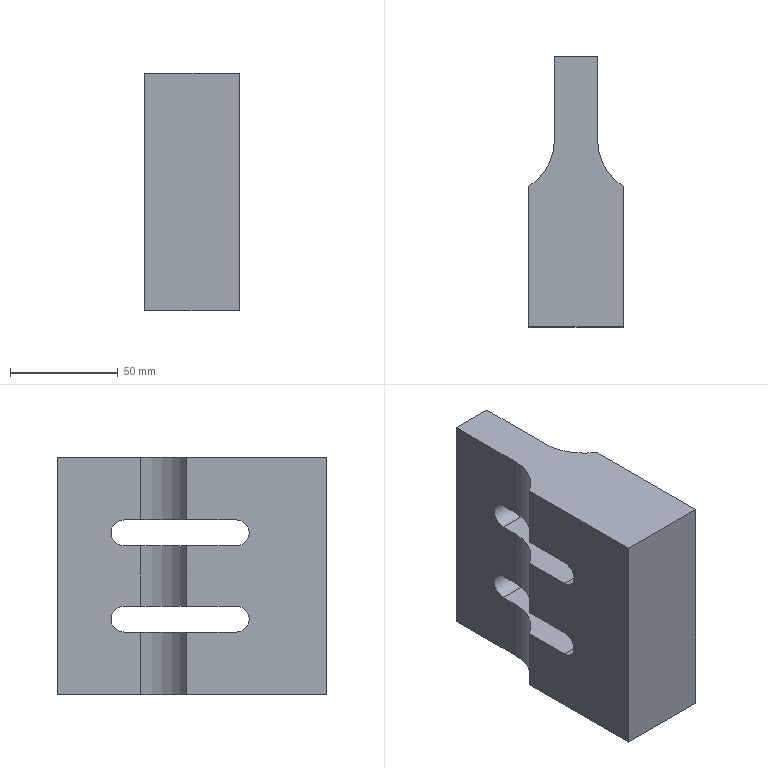Component | SolidWorks | Assembly4.1-1_113.1-1 | 1 solid | 22 faces | box 44 x 125 x 110 mm | volume 414066 mm3 | plane 12 | cylinder 10 | commonest cylinder face diameters 50 x6 12 x4
build123d program:
from build123d import *

# Parameters (mm, degrees)
SKETCH1_W           = 110
SKETCH1_H           = 125
BOSS_EXTRUDE1_DEPTH = 22
CUT_EXTRUDE1_DEPTH  = 124
CUT_EXTRUDE2_DEPTH  = 62


with BuildPart() as part:
    # Sketch1 → Boss-Extrude1 (new, symmetric)
    with BuildSketch(Plane.XY):
        Rectangle(SKETCH1_W, SKETCH1_H)
    extrude(amount=BOSS_EXTRUDE1_DEPTH, both=True)

    # Sketch2 → Cut-Extrude1 (cut)
    with BuildSketch(Plane(origin=(55, 0, 0), x_dir=(0, 0, -1), z_dir=(1, 0, 0))):
        with BuildLine():
            Line((-22, 2.5), (-46.846, 2.5))
            Line((-46.846, 2.5), (-46.846, 62.5))
            Line((-46.846, 62.5), (-10, 62.5))
            Line((-10, 62.5), (-10, 23.854))
            ThreePointArc((-10, 23.854), (-13.206, 11.607), (-22, 2.5))
        make_face()
        with BuildLine():
            Line((46.846, 62.5), (10, 62.5))
            Line((10, 62.5), (10, 23.854))
            ThreePointArc((10, 23.854), (13.206, 11.607), (22, 2.5))
            Line((22, 2.5), (46.846, 2.5))
            Line((46.846, 2.5), (46.846, 62.5))
        make_face()
    extrude(amount=-CUT_EXTRUDE1_DEPTH, mode=Mode.SUBTRACT)

    # Sketch3 → Cut-Extrude2 (cut, symmetric)
    with BuildSketch(Plane.XY):
        with BuildLine():
            Line((-14, 31.5), (-14, -20.5))
            ThreePointArc((-14, -20.5), (-20, -26.5), (-26, -20.5))
            Line((-26, -20.5), (-26, 31.5))
            ThreePointArc((-26, 31.5), (-20, 37.5), (-14, 31.5))
        make_face()
        with BuildLine():
            Line((26, 31.5), (26, -20.5))
            ThreePointArc((26, -20.5), (20, -26.5), (14, -20.5))
            Line((14, -20.5), (14, 31.5))
            ThreePointArc((14, 31.5), (20, 37.5), (26, 31.5))
        make_face()
    extrude(amount=CUT_EXTRUDE2_DEPTH, both=True, mode=Mode.SUBTRACT)


solid = part.part

# Placed as in the assembly
solid = solid.moved(Location((0, 88, -0.4), (0, 90, 0)))
STEP:
#1=COLOUR_RGB('',0.7922,0.8196,0.9333);
#2=FILL_AREA_STYLE_COLOUR('',#1);
#3=FILL_AREA_STYLE('',(#2));
#4=SURFACE_STYLE_FILL_AREA(#3);
#5=SURFACE_SIDE_STYLE('',(#4));
#6=SURFACE_STYLE_USAGE(.BOTH.,#5);
#7=PRESENTATION_STYLE_ASSIGNMENT((#6));
#8=CARTESIAN_POINT('',(-0.3937,4.404,1.008));
#9=VERTEX_POINT('',#8);
#10=CARTESIAN_POINT('',(-0.3937,4.404,2.15));
#11=VERTEX_POINT('',#10);
#12=CARTESIAN_POINT('',(-0.3937,4.404,-2.732));
#13=DIRECTION('',(-0.,0.,1.));
#14=VECTOR('',#13,39.37);
#15=LINE('',#12,#14);
#16=EDGE_CURVE('',#9,#11,#15,.T.);
#17=ORIENTED_EDGE('',*,*,#16,.F.);
#18=CARTESIAN_POINT('',(-0.8661,3.563,1.008));
#19=VERTEX_POINT('',#18);
#20=CARTESIAN_POINT('',(-1.378,4.404,1.008));
#21=DIRECTION('',(0.,-0.,-1.));
#22=DIRECTION('',(0.,1.,-0.));
#23=AXIS2_PLACEMENT_3D('',#20,#21,#22);
#24=CIRCLE('',#23,0.9843);
#25=EDGE_CURVE('',#9,#19,#24,.T.);
#26=ORIENTED_EDGE('',*,*,#25,.T.);
#27=CARTESIAN_POINT('',(-0.8661,3.563,2.15));
#28=VERTEX_POINT('',#27);
#29=CARTESIAN_POINT('',(-0.8661,3.563,2.15));
#30=DIRECTION('',(-0.,0.,1.));
#31=VECTOR('',#30,39.37);
#32=LINE('',#29,#31);
#33=EDGE_CURVE('',#19,#28,#32,.T.);
#34=ORIENTED_EDGE('',*,*,#33,.T.);
#35=CARTESIAN_POINT('',(-1.378,4.404,2.15));
#36=DIRECTION('',(-0.,0.,1.));
#37=DIRECTION('',(0.,-1.,0.));
#38=AXIS2_PLACEMENT_3D('',#35,#36,#37);
#39=CIRCLE('',#38,0.9843);
#40=EDGE_CURVE('',#28,#11,#39,.T.);
#41=ORIENTED_EDGE('',*,*,#40,.T.);
#42=EDGE_LOOP('',(#17,#26,#34,#41));
#43=FACE_OUTER_BOUND('',#42,.T.);
#44=CARTESIAN_POINT('',(-1.378,4.404,-2.732));
#45=DIRECTION('',(-0.,0.,1.));
#46=DIRECTION('',(0.,1.,0.));
#47=AXIS2_PLACEMENT_3D('',#44,#45,#46);
#48=CYLINDRICAL_SURFACE('',#47,0.9843);
#49=ADVANCED_FACE('',(#43),#48,.F.);
#50=CARTESIAN_POINT('',(0.8661,3.563,1.008));
#51=VERTEX_POINT('',#50);
#52=CARTESIAN_POINT('',(0.8661,3.563,2.15));
#53=VERTEX_POINT('',#52);
#54=CARTESIAN_POINT('',(0.8661,3.563,-2.732));
#55=DIRECTION('',(-0.,0.,1.));
#56=VECTOR('',#55,39.37);
#57=LINE('',#54,#56);
#58=EDGE_CURVE('',#51,#53,#57,.T.);
#59=ORIENTED_EDGE('',*,*,#58,.F.);
#60=CARTESIAN_POINT('',(0.3937,4.404,1.008));
#61=VERTEX_POINT('',#60);
#62=CARTESIAN_POINT('',(1.378,4.404,1.008));
#63=DIRECTION('',(0.,-0.,-1.));
#64=DIRECTION('',(0.,1.,-0.));
#65=AXIS2_PLACEMENT_3D('',#62,#63,#64);
#66=CIRCLE('',#65,0.9843);
#67=EDGE_CURVE('',#51,#61,#66,.T.);
#68=ORIENTED_EDGE('',*,*,#67,.T.);
#69=CARTESIAN_POINT('',(0.3937,4.404,2.15));
#70=VERTEX_POINT('',#69);
#71=CARTESIAN_POINT('',(0.3937,4.404,-2.732));
#72=DIRECTION('',(-0.,0.,1.));
#73=VECTOR('',#72,39.37);
#74=LINE('',#71,#73);
#75=EDGE_CURVE('',#61,#70,#74,.T.);
#76=ORIENTED_EDGE('',*,*,#75,.T.);
#77=CARTESIAN_POINT('',(1.378,4.404,2.15));
#78=DIRECTION('',(-0.,0.,1.));
#79=DIRECTION('',(0.,1.,0.));
#80=AXIS2_PLACEMENT_3D('',#77,#78,#79);
#81=CIRCLE('',#80,0.9843);
#82=EDGE_CURVE('',#70,#53,#81,.T.);
#83=ORIENTED_EDGE('',*,*,#82,.T.);
#84=EDGE_LOOP('',(#59,#68,#76,#83));
#85=FACE_OUTER_BOUND('',#84,.T.);
#86=CARTESIAN_POINT('',(1.378,4.404,-2.732));
#87=DIRECTION('',(-0.,0.,1.));
#88=DIRECTION('',(0.,1.,0.));
#89=AXIS2_PLACEMENT_3D('',#86,#87,#88);
#90=CYLINDRICAL_SURFACE('',#89,0.9843);
#91=ADVANCED_FACE('',(#85),#90,.F.);
#92=CARTESIAN_POINT('',(-0.8661,3.563,-0.5669));
#93=VERTEX_POINT('',#92);
#94=CARTESIAN_POINT('',(-0.8661,3.563,0.5354));
#95=VERTEX_POINT('',#94);
#96=CARTESIAN_POINT('',(-0.8661,3.563,2.15));
#97=DIRECTION('',(-0.,0.,1.));
#98=VECTOR('',#97,39.37);
#99=LINE('',#96,#98);
#100=EDGE_CURVE('',#93,#95,#99,.T.);
#101=ORIENTED_EDGE('',*,*,#100,.T.);
#102=CARTESIAN_POINT('',(-0.3937,4.404,0.5354));
#103=VERTEX_POINT('',#102);
#104=CARTESIAN_POINT('',(-1.378,4.404,0.5354));
#105=DIRECTION('',(-0.,0.,1.));
#106=DIRECTION('',(0.,-1.,0.));
#107=AXIS2_PLACEMENT_3D('',#104,#105,#106);
#108=CIRCLE('',#107,0.9843);
#109=EDGE_CURVE('',#95,#103,#108,.T.);
#110=ORIENTED_EDGE('',*,*,#109,.T.);
#111=CARTESIAN_POINT('',(-0.3937,4.404,-0.5669));
#112=VERTEX_POINT('',#111);
#113=CARTESIAN_POINT('',(-0.3937,4.404,-2.732));
#114=DIRECTION('',(-0.,0.,1.));
#115=VECTOR('',#114,39.37);
#116=LINE('',#113,#115);
#117=EDGE_CURVE('',#112,#103,#116,.T.);
#118=ORIENTED_EDGE('',*,*,#117,.F.);
#119=CARTESIAN_POINT('',(-1.378,4.404,-0.5669));
#120=DIRECTION('',(0.,-0.,-1.));
#121=DIRECTION('',(1.,0.,0.));
#122=AXIS2_PLACEMENT_3D('',#119,#120,#121);
#123=CIRCLE('',#122,0.9843);
#124=EDGE_CURVE('',#112,#93,#123,.T.);
#125=ORIENTED_EDGE('',*,*,#124,.T.);
#126=EDGE_LOOP('',(#101,#110,#118,#125));
#127=FACE_OUTER_BOUND('',#126,.T.);
#128=CARTESIAN_POINT('',(-1.378,4.404,-2.732));
#129=DIRECTION('',(-0.,0.,1.));
#130=DIRECTION('',(0.,1.,0.));
#131=AXIS2_PLACEMENT_3D('',#128,#129,#130);
#132=CYLINDRICAL_SURFACE('',#131,0.9843);
#133=ADVANCED_FACE('',(#127),#132,.F.);
#134=CARTESIAN_POINT('',(0.3937,4.404,-0.5669));
#135=VERTEX_POINT('',#134);
#136=CARTESIAN_POINT('',(0.3937,4.404,0.5354));
#137=VERTEX_POINT('',#136);
#138=CARTESIAN_POINT('',(0.3937,4.404,-2.732));
#139=DIRECTION('',(-0.,0.,1.));
#140=VECTOR('',#139,39.37);
#141=LINE('',#138,#140);
#142=EDGE_CURVE('',#135,#137,#141,.T.);
#143=ORIENTED_EDGE('',*,*,#142,.T.);
#144=CARTESIAN_POINT('',(0.8661,3.563,0.5354));
#145=VERTEX_POINT('',#144);
#146=CARTESIAN_POINT('',(1.378,4.404,0.5354));
#147=DIRECTION('',(-0.,0.,1.));
#148=DIRECTION('',(-0.,-1.,0.));
#149=AXIS2_PLACEMENT_3D('',#146,#147,#148);
#150=CIRCLE('',#149,0.9843);
#151=EDGE_CURVE('',#137,#145,#150,.T.);
#152=ORIENTED_EDGE('',*,*,#151,.T.);
#153=CARTESIAN_POINT('',(0.8661,3.563,-0.5669));
#154=VERTEX_POINT('',#153);
#155=CARTESIAN_POINT('',(0.8661,3.563,-2.732));
#156=DIRECTION('',(-0.,0.,1.));
#157=VECTOR('',#156,39.37);
#158=LINE('',#155,#157);
#159=EDGE_CURVE('',#154,#145,#158,.T.);
#160=ORIENTED_EDGE('',*,*,#159,.F.);
#161=CARTESIAN_POINT('',(1.378,4.404,-0.5669));
#162=DIRECTION('',(0.,-0.,-1.));
#163=DIRECTION('',(1.,0.,0.));
#164=AXIS2_PLACEMENT_3D('',#161,#162,#163);
#165=CIRCLE('',#164,0.9843);
#166=EDGE_CURVE('',#154,#135,#165,.T.);
#167=ORIENTED_EDGE('',*,*,#166,.T.);
#168=EDGE_LOOP('',(#143,#152,#160,#167));
#169=FACE_OUTER_BOUND('',#168,.T.);
#170=CARTESIAN_POINT('',(1.378,4.404,-2.732));
#171=DIRECTION('',(-0.,0.,1.));
#172=DIRECTION('',(0.,1.,0.));
#173=AXIS2_PLACEMENT_3D('',#170,#171,#172);
#174=CYLINDRICAL_SURFACE('',#173,0.9843);
#175=ADVANCED_FACE('',(#169),#174,.F.);
#176=ORIENTED_EDGE('',*,*,#82,.F.);
#177=CARTESIAN_POINT('',(0.3937,5.925,2.15));
#178=VERTEX_POINT('',#177);
#179=CARTESIAN_POINT('',(0.3937,5.925,2.15));
#180=DIRECTION('',(-0.,-1.,0.));
#181=VECTOR('',#180,39.37);
#182=LINE('',#179,#181);
#183=EDGE_CURVE('',#178,#70,#182,.T.);
#184=ORIENTED_EDGE('',*,*,#183,.F.);
#185=CARTESIAN_POINT('',(-0.3937,5.925,2.15));
#186=VERTEX_POINT('',#185);
#187=CARTESIAN_POINT('',(-0.8661,5.925,2.15));
#188=DIRECTION('',(1.,-0.,0.));
#189=VECTOR('',#188,39.37);
#190=LINE('',#187,#189);
#191=EDGE_CURVE('',#186,#178,#190,.T.);
#192=ORIENTED_EDGE('',*,*,#191,.F.);
#193=CARTESIAN_POINT('',(-0.3937,5.925,2.15));
#194=DIRECTION('',(-0.,1.,-0.));
#195=VECTOR('',#194,39.37);
#196=LINE('',#193,#195);
#197=EDGE_CURVE('',#11,#186,#196,.T.);
#198=ORIENTED_EDGE('',*,*,#197,.F.);
#199=ORIENTED_EDGE('',*,*,#40,.F.);
#200=CARTESIAN_POINT('',(-0.8661,1.004,2.15));
#201=VERTEX_POINT('',#200);
#202=CARTESIAN_POINT('',(-0.8661,5.925,2.15));
#203=DIRECTION('',(0.,1.,-0.));
#204=VECTOR('',#203,39.37);
#205=LINE('',#202,#204);
#206=EDGE_CURVE('',#201,#28,#205,.T.);
#207=ORIENTED_EDGE('',*,*,#206,.F.);
#208=CARTESIAN_POINT('',(0.8661,1.004,2.15));
#209=VERTEX_POINT('',#208);
#210=CARTESIAN_POINT('',(-0.8661,1.004,2.15));
#211=DIRECTION('',(1.,-0.,0.));
#212=VECTOR('',#211,39.37);
#213=LINE('',#210,#212);
#214=EDGE_CURVE('',#201,#209,#213,.T.);
#215=ORIENTED_EDGE('',*,*,#214,.T.);
#216=CARTESIAN_POINT('',(0.8661,5.925,2.15));
#217=DIRECTION('',(0.,1.,-0.));
#218=VECTOR('',#217,39.37);
#219=LINE('',#216,#218);
#220=EDGE_CURVE('',#209,#53,#219,.T.);
#221=ORIENTED_EDGE('',*,*,#220,.T.);
#222=EDGE_LOOP('',(#176,#184,#192,#198,#199,#207,#215,#221));
#223=FACE_OUTER_BOUND('',#222,.T.);
#224=CARTESIAN_POINT('',(-0.8661,5.925,2.15));
#225=DIRECTION('',(0.,-0.,-1.));
#226=DIRECTION('',(-0.,-1.,0.));
#227=AXIS2_PLACEMENT_3D('',#224,#225,#226);
#228=PLANE('',#227);
#229=ADVANCED_FACE('',(#223),#228,.F.);
#230=ORIENTED_EDGE('',*,*,#191,.T.);
#231=CARTESIAN_POINT('',(0.3937,5.925,-2.181));
#232=VERTEX_POINT('',#231);
#233=CARTESIAN_POINT('',(0.3937,5.925,-2.732));
#234=DIRECTION('',(-0.,0.,1.));
#235=VECTOR('',#234,39.37);
#236=LINE('',#233,#235);
#237=EDGE_CURVE('',#232,#178,#236,.T.);
#238=ORIENTED_EDGE('',*,*,#237,.F.);
#239=CARTESIAN_POINT('',(-0.3937,5.925,-2.181));
#240=VERTEX_POINT('',#239);
#241=CARTESIAN_POINT('',(-0.8661,5.925,-2.181));
#242=DIRECTION('',(1.,-0.,0.));
#243=VECTOR('',#242,39.37);
#244=LINE('',#241,#243);
#245=EDGE_CURVE('',#240,#232,#244,.T.);
#246=ORIENTED_EDGE('',*,*,#245,.F.);
#247=CARTESIAN_POINT('',(-0.3937,5.925,-2.732));
#248=DIRECTION('',(-0.,0.,1.));
#249=VECTOR('',#248,39.37);
#250=LINE('',#247,#249);
#251=EDGE_CURVE('',#240,#186,#250,.T.);
#252=ORIENTED_EDGE('',*,*,#251,.T.);
#253=EDGE_LOOP('',(#230,#238,#246,#252));
#254=FACE_OUTER_BOUND('',#253,.T.);
#255=CARTESIAN_POINT('',(-0.8661,5.925,-2.181));
#256=DIRECTION('',(-0.,-1.,0.));
#257=DIRECTION('',(1.,-0.,0.));
#258=AXIS2_PLACEMENT_3D('',#255,#256,#257);
#259=PLANE('',#258);
#260=ADVANCED_FACE('',(#254),#259,.F.);
#261=ORIENTED_EDGE('',*,*,#245,.T.);
#262=CARTESIAN_POINT('',(0.3937,4.404,-2.181));
#263=VERTEX_POINT('',#262);
#264=CARTESIAN_POINT('',(0.3937,5.925,-2.181));
#265=DIRECTION('',(-0.,-1.,0.));
#266=VECTOR('',#265,39.37);
#267=LINE('',#264,#266);
#268=EDGE_CURVE('',#232,#263,#267,.T.);
#269=ORIENTED_EDGE('',*,*,#268,.T.);
#270=CARTESIAN_POINT('',(0.8661,3.563,-2.181));
#271=VERTEX_POINT('',#270);
#272=CARTESIAN_POINT('',(1.378,4.404,-2.181));
#273=DIRECTION('',(-0.,0.,1.));
#274=DIRECTION('',(0.,1.,-0.));
#275=AXIS2_PLACEMENT_3D('',#272,#273,#274);
#276=CIRCLE('',#275,0.9843);
#277=EDGE_CURVE('',#263,#271,#276,.T.);
#278=ORIENTED_EDGE('',*,*,#277,.T.);
#279=CARTESIAN_POINT('',(0.8661,1.004,-2.181));
#280=VERTEX_POINT('',#279);
#281=CARTESIAN_POINT('',(0.8661,5.925,-2.181));
#282=DIRECTION('',(-0.,-1.,0.));
#283=VECTOR('',#282,39.37);
#284=LINE('',#281,#283);
#285=EDGE_CURVE('',#271,#280,#284,.T.);
#286=ORIENTED_EDGE('',*,*,#285,.T.);
#287=CARTESIAN_POINT('',(-0.8661,1.004,-2.181));
#288=VERTEX_POINT('',#287);
#289=CARTESIAN_POINT('',(-0.8661,1.004,-2.181));
#290=DIRECTION('',(1.,-0.,0.));
#291=VECTOR('',#290,39.37);
#292=LINE('',#289,#291);
#293=EDGE_CURVE('',#288,#280,#292,.T.);
#294=ORIENTED_EDGE('',*,*,#293,.F.);
#295=CARTESIAN_POINT('',(-0.8661,3.563,-2.181));
#296=VERTEX_POINT('',#295);
#297=CARTESIAN_POINT('',(-0.8661,5.925,-2.181));
#298=DIRECTION('',(-0.,-1.,0.));
#299=VECTOR('',#298,39.37);
#300=LINE('',#297,#299);
#301=EDGE_CURVE('',#296,#288,#300,.T.);
#302=ORIENTED_EDGE('',*,*,#301,.F.);
#303=CARTESIAN_POINT('',(-0.3937,4.404,-2.181));
#304=VERTEX_POINT('',#303);
#305=CARTESIAN_POINT('',(-1.378,4.404,-2.181));
#306=DIRECTION('',(-0.,0.,1.));
#307=DIRECTION('',(0.,1.,-0.));
#308=AXIS2_PLACEMENT_3D('',#305,#306,#307);
#309=CIRCLE('',#308,0.9843);
#310=EDGE_CURVE('',#296,#304,#309,.T.);
#311=ORIENTED_EDGE('',*,*,#310,.T.);
#312=CARTESIAN_POINT('',(-0.3937,5.925,-2.181));
#313=DIRECTION('',(-0.,1.,-0.));
#314=VECTOR('',#313,39.37);
#315=LINE('',#312,#314);
#316=EDGE_CURVE('',#304,#240,#315,.T.);
#317=ORIENTED_EDGE('',*,*,#316,.T.);
#318=EDGE_LOOP('',(#261,#269,#278,#286,#294,#302,#311,#317));
#319=FACE_OUTER_BOUND('',#318,.T.);
#320=CARTESIAN_POINT('',(-0.8661,5.925,-2.181));
#321=DIRECTION('',(-0.,0.,1.));
#322=DIRECTION('',(0.,1.,-0.));
#323=AXIS2_PLACEMENT_3D('',#320,#321,#322);
#324=PLANE('',#323);
#325=ADVANCED_FACE('',(#319),#324,.F.);
#326=CARTESIAN_POINT('',(0.8661,1.004,-2.181));
#327=DIRECTION('',(-0.,0.,1.));
#328=VECTOR('',#327,39.37);
#329=LINE('',#326,#328);
#330=EDGE_CURVE('',#280,#209,#329,.T.);
#331=ORIENTED_EDGE('',*,*,#330,.T.);
#332=ORIENTED_EDGE('',*,*,#214,.F.);
#333=CARTESIAN_POINT('',(-0.8661,1.004,-2.181));
#334=DIRECTION('',(-0.,0.,1.));
#335=VECTOR('',#334,39.37);
#336=LINE('',#333,#335);
#337=EDGE_CURVE('',#288,#201,#336,.T.);
#338=ORIENTED_EDGE('',*,*,#337,.F.);
#339=ORIENTED_EDGE('',*,*,#293,.T.);
#340=EDGE_LOOP('',(#331,#332,#338,#339));
#341=FACE_OUTER_BOUND('',#340,.T.);
#342=CARTESIAN_POINT('',(-0.8661,1.004,-2.181));
#343=DIRECTION('',(0.,1.,-0.));
#344=DIRECTION('',(-1.,0.,-0.));
#345=AXIS2_PLACEMENT_3D('',#342,#343,#344);
#346=PLANE('',#345);
#347=ADVANCED_FACE('',(#341),#346,.F.);
#348=CARTESIAN_POINT('',(-0.8661,2.657,1.008));
#349=VERTEX_POINT('',#348);
#350=CARTESIAN_POINT('',(-0.8661,1.004,1.008));
#351=DIRECTION('',(0.,1.,-0.));
#352=VECTOR('',#351,39.37);
#353=LINE('',#350,#352);
#354=EDGE_CURVE('',#349,#19,#353,.T.);
#355=ORIENTED_EDGE('',*,*,#354,.F.);
#356=CARTESIAN_POINT('',(-0.8661,2.657,0.5354));
#357=VERTEX_POINT('',#356);
#358=CARTESIAN_POINT('',(-0.8661,2.657,0.7717));
#359=DIRECTION('',(-1.,0.,-0.));
#360=DIRECTION('',(0.,0.,1.));
#361=AXIS2_PLACEMENT_3D('',#358,#359,#360);
#362=CIRCLE('',#361,0.2362);
#363=EDGE_CURVE('',#357,#349,#362,.T.);
#364=ORIENTED_EDGE('',*,*,#363,.F.);
#365=CARTESIAN_POINT('',(-0.8661,1.004,0.5354));
#366=DIRECTION('',(-0.,-1.,0.));
#367=VECTOR('',#366,39.37);
#368=LINE('',#365,#367);
#369=EDGE_CURVE('',#95,#357,#368,.T.);
#370=ORIENTED_EDGE('',*,*,#369,.F.);
#371=ORIENTED_EDGE('',*,*,#100,.F.);
#372=CARTESIAN_POINT('',(-0.8661,2.657,-0.5669));
#373=VERTEX_POINT('',#372);
#374=CARTESIAN_POINT('',(-0.8661,1.004,-0.5669));
#375=DIRECTION('',(0.,1.,-0.));
#376=VECTOR('',#375,39.37);
#377=LINE('',#374,#376);
#378=EDGE_CURVE('',#373,#93,#377,.T.);
#379=ORIENTED_EDGE('',*,*,#378,.F.);
#380=CARTESIAN_POINT('',(-0.8661,2.657,-1.039));
#381=VERTEX_POINT('',#380);
#382=CARTESIAN_POINT('',(-0.8661,2.657,-0.8031));
#383=DIRECTION('',(-1.,0.,-0.));
#384=DIRECTION('',(0.,0.,1.));
#385=AXIS2_PLACEMENT_3D('',#382,#383,#384);
#386=CIRCLE('',#385,0.2362);
#387=EDGE_CURVE('',#381,#373,#386,.T.);
#388=ORIENTED_EDGE('',*,*,#387,.F.);
#389=CARTESIAN_POINT('',(-0.8661,3.563,-1.039));
#390=VERTEX_POINT('',#389);
#391=CARTESIAN_POINT('',(-0.8661,1.004,-1.039));
#392=DIRECTION('',(-0.,-1.,0.));
#393=VECTOR('',#392,39.37);
#394=LINE('',#391,#393);
#395=EDGE_CURVE('',#390,#381,#394,.T.);
#396=ORIENTED_EDGE('',*,*,#395,.F.);
#397=CARTESIAN_POINT('',(-0.8661,3.563,2.15));
#398=DIRECTION('',(-0.,0.,1.));
#399=VECTOR('',#398,39.37);
#400=LINE('',#397,#399);
#401=EDGE_CURVE('',#296,#390,#400,.T.);
#402=ORIENTED_EDGE('',*,*,#401,.F.);
#403=ORIENTED_EDGE('',*,*,#301,.T.);
#404=ORIENTED_EDGE('',*,*,#337,.T.);
#405=ORIENTED_EDGE('',*,*,#206,.T.);
#406=ORIENTED_EDGE('',*,*,#33,.F.);
#407=EDGE_LOOP('',(#355,#364,#370,#371,#379,#388,#396,#402,#403,#404,#405,#406));
#408=FACE_OUTER_BOUND('',#407,.T.);
#409=CARTESIAN_POINT('',(-0.8661,1.004,2.15));
#410=DIRECTION('',(-1.,0.,-0.));
#411=DIRECTION('',(-0.,0.,1.));
#412=AXIS2_PLACEMENT_3D('',#409,#410,#411);
#413=PLANE('',#412);
#414=ADVANCED_FACE('',(#408),#413,.T.);
#415=CARTESIAN_POINT('',(0.8661,2.657,0.5354));
#416=VERTEX_POINT('',#415);
#417=CARTESIAN_POINT('',(0.8661,2.657,1.008));
#418=VERTEX_POINT('',#417);
#419=CARTESIAN_POINT('',(0.8661,2.657,0.7717));
#420=DIRECTION('',(-1.,0.,-0.));
#421=DIRECTION('',(0.,0.,1.));
#422=AXIS2_PLACEMENT_3D('',#419,#420,#421);
#423=CIRCLE('',#422,0.2362);
#424=EDGE_CURVE('',#416,#418,#423,.T.);
#425=ORIENTED_EDGE('',*,*,#424,.T.);
#426=CARTESIAN_POINT('',(0.8661,1.004,1.008));
#427=DIRECTION('',(0.,1.,-0.));
#428=VECTOR('',#427,39.37);
#429=LINE('',#426,#428);
#430=EDGE_CURVE('',#418,#51,#429,.T.);
#431=ORIENTED_EDGE('',*,*,#430,.T.);
#432=ORIENTED_EDGE('',*,*,#58,.T.);
#433=ORIENTED_EDGE('',*,*,#220,.F.);
#434=ORIENTED_EDGE('',*,*,#330,.F.);
#435=ORIENTED_EDGE('',*,*,#285,.F.);
#436=CARTESIAN_POINT('',(0.8661,3.563,-1.039));
#437=VERTEX_POINT('',#436);
#438=CARTESIAN_POINT('',(0.8661,3.563,-2.732));
#439=DIRECTION('',(-0.,0.,1.));
#440=VECTOR('',#439,39.37);
#441=LINE('',#438,#440);
#442=EDGE_CURVE('',#271,#437,#441,.T.);
#443=ORIENTED_EDGE('',*,*,#442,.T.);
#444=CARTESIAN_POINT('',(0.8661,2.657,-1.039));
#445=VERTEX_POINT('',#444);
#446=CARTESIAN_POINT('',(0.8661,1.004,-1.039));
#447=DIRECTION('',(-0.,-1.,0.));
#448=VECTOR('',#447,39.37);
#449=LINE('',#446,#448);
#450=EDGE_CURVE('',#437,#445,#449,.T.);
#451=ORIENTED_EDGE('',*,*,#450,.T.);
#452=CARTESIAN_POINT('',(0.8661,2.657,-0.5669));
#453=VERTEX_POINT('',#452);
#454=CARTESIAN_POINT('',(0.8661,2.657,-0.8031));
#455=DIRECTION('',(-1.,0.,-0.));
#456=DIRECTION('',(0.,0.,1.));
#457=AXIS2_PLACEMENT_3D('',#454,#455,#456);
#458=CIRCLE('',#457,0.2362);
#459=EDGE_CURVE('',#445,#453,#458,.T.);
#460=ORIENTED_EDGE('',*,*,#459,.T.);
#461=CARTESIAN_POINT('',(0.8661,1.004,-0.5669));
#462=DIRECTION('',(0.,1.,-0.));
#463=VECTOR('',#462,39.37);
#464=LINE('',#461,#463);
#465=EDGE_CURVE('',#453,#154,#464,.T.);
#466=ORIENTED_EDGE('',*,*,#465,.T.);
#467=ORIENTED_EDGE('',*,*,#159,.T.);
#468=CARTESIAN_POINT('',(0.8661,1.004,0.5354));
#469=DIRECTION('',(-0.,-1.,0.));
#470=VECTOR('',#469,39.37);
#471=LINE('',#468,#470);
#472=EDGE_CURVE('',#145,#416,#471,.T.);
#473=ORIENTED_EDGE('',*,*,#472,.T.);
#474=EDGE_LOOP('',(#425,#431,#432,#433,#434,#435,#443,#451,#460,#466,#467,#473));
#475=FACE_OUTER_BOUND('',#474,.T.);
#476=CARTESIAN_POINT('',(0.8661,1.004,2.15));
#477=DIRECTION('',(-1.,0.,-0.));
#478=DIRECTION('',(-0.,0.,1.));
#479=AXIS2_PLACEMENT_3D('',#476,#477,#478);
#480=PLANE('',#479);
#481=ADVANCED_FACE('',(#475),#480,.F.);
#482=CARTESIAN_POINT('',(-0.3937,4.705,0.5354));
#483=VERTEX_POINT('',#482);
#484=CARTESIAN_POINT('',(-0.3937,4.705,1.008));
#485=VERTEX_POINT('',#484);
#486=CARTESIAN_POINT('',(-0.3937,4.705,0.7717));
#487=DIRECTION('',(1.,0.,0.));
#488=DIRECTION('',(0.,1.,0.));
#489=AXIS2_PLACEMENT_3D('',#486,#487,#488);
#490=CIRCLE('',#489,0.2362);
#491=EDGE_CURVE('',#483,#485,#490,.T.);
#492=ORIENTED_EDGE('',*,*,#491,.T.);
#493=CARTESIAN_POINT('',(-0.3937,5.925,1.008));
#494=DIRECTION('',(0.,-1.,0.));
#495=VECTOR('',#494,39.37);
#496=LINE('',#493,#495);
#497=EDGE_CURVE('',#485,#9,#496,.T.);
#498=ORIENTED_EDGE('',*,*,#497,.T.);
#499=ORIENTED_EDGE('',*,*,#16,.T.);
#500=ORIENTED_EDGE('',*,*,#197,.T.);
#501=ORIENTED_EDGE('',*,*,#251,.F.);
#502=ORIENTED_EDGE('',*,*,#316,.F.);
#503=CARTESIAN_POINT('',(-0.3937,4.404,-1.039));
#504=VERTEX_POINT('',#503);
#505=CARTESIAN_POINT('',(-0.3937,4.404,-2.732));
#506=DIRECTION('',(-0.,0.,1.));
#507=VECTOR('',#506,39.37);
#508=LINE('',#505,#507);
#509=EDGE_CURVE('',#304,#504,#508,.T.);
#510=ORIENTED_EDGE('',*,*,#509,.T.);
#511=CARTESIAN_POINT('',(-0.3937,4.705,-1.039));
#512=VERTEX_POINT('',#511);
#513=CARTESIAN_POINT('',(-0.3937,5.925,-1.039));
#514=DIRECTION('',(-0.,1.,-0.));
#515=VECTOR('',#514,39.37);
#516=LINE('',#513,#515);
#517=EDGE_CURVE('',#504,#512,#516,.T.);
#518=ORIENTED_EDGE('',*,*,#517,.T.);
#519=CARTESIAN_POINT('',(-0.3937,4.705,-0.5669));
#520=VERTEX_POINT('',#519);
#521=CARTESIAN_POINT('',(-0.3937,4.705,-0.8031));
#522=DIRECTION('',(1.,0.,0.));
#523=DIRECTION('',(0.,1.,0.));
#524=AXIS2_PLACEMENT_3D('',#521,#522,#523);
#525=CIRCLE('',#524,0.2362);
#526=EDGE_CURVE('',#512,#520,#525,.T.);
#527=ORIENTED_EDGE('',*,*,#526,.T.);
#528=CARTESIAN_POINT('',(-0.3937,5.925,-0.5669));
#529=DIRECTION('',(0.,-1.,0.));
#530=VECTOR('',#529,39.37);
#531=LINE('',#528,#530);
#532=EDGE_CURVE('',#520,#112,#531,.T.);
#533=ORIENTED_EDGE('',*,*,#532,.T.);
#534=ORIENTED_EDGE('',*,*,#117,.T.);
#535=CARTESIAN_POINT('',(-0.3937,5.925,0.5354));
#536=DIRECTION('',(-0.,1.,-0.));
#537=VECTOR('',#536,39.37);
#538=LINE('',#535,#537);
#539=EDGE_CURVE('',#103,#483,#538,.T.);
#540=ORIENTED_EDGE('',*,*,#539,.T.);
#541=EDGE_LOOP('',(#492,#498,#499,#500,#501,#502,#510,#518,#527,#533,#534,#540));
#542=FACE_OUTER_BOUND('',#541,.T.);
#543=CARTESIAN_POINT('',(-0.3937,5.925,-2.732));
#544=DIRECTION('',(1.,0.,0.));
#545=DIRECTION('',(-0.,1.,-0.));
#546=AXIS2_PLACEMENT_3D('',#543,#544,#545);
#547=PLANE('',#546);
#548=ADVANCED_FACE('',(#542),#547,.F.);
#549=ORIENTED_EDGE('',*,*,#401,.T.);
#550=CARTESIAN_POINT('',(-1.378,4.404,-1.039));
#551=DIRECTION('',(-0.,0.,1.));
#552=DIRECTION('',(0.,-1.,0.));
#553=AXIS2_PLACEMENT_3D('',#550,#551,#552);
#554=CIRCLE('',#553,0.9843);
#555=EDGE_CURVE('',#390,#504,#554,.T.);
#556=ORIENTED_EDGE('',*,*,#555,.T.);
#557=ORIENTED_EDGE('',*,*,#509,.F.);
#558=ORIENTED_EDGE('',*,*,#310,.F.);
#559=EDGE_LOOP('',(#549,#556,#557,#558));
#560=FACE_OUTER_BOUND('',#559,.T.);
#561=CARTESIAN_POINT('',(-1.378,4.404,-2.732));
#562=DIRECTION('',(-0.,0.,1.));
#563=DIRECTION('',(0.,1.,0.));
#564=AXIS2_PLACEMENT_3D('',#561,#562,#563);
#565=CYLINDRICAL_SURFACE('',#564,0.9843);
#566=ADVANCED_FACE('',(#560),#565,.F.);
#567=ORIENTED_EDGE('',*,*,#75,.F.);
#568=CARTESIAN_POINT('',(0.3937,4.705,1.008));
#569=VERTEX_POINT('',#568);
#570=CARTESIAN_POINT('',(0.3937,5.925,1.008));
#571=DIRECTION('',(0.,1.,-0.));
#572=VECTOR('',#571,39.37);
#573=LINE('',#570,#572);
#574=EDGE_CURVE('',#61,#569,#573,.T.);
#575=ORIENTED_EDGE('',*,*,#574,.T.);
#576=CARTESIAN_POINT('',(0.3937,4.705,0.5354));
#577=VERTEX_POINT('',#576);
#578=CARTESIAN_POINT('',(0.3937,4.705,0.7717));
#579=DIRECTION('',(-1.,0.,-0.));
#580=DIRECTION('',(-0.,-1.,0.));
#581=AXIS2_PLACEMENT_3D('',#578,#579,#580);
#582=CIRCLE('',#581,0.2362);
#583=EDGE_CURVE('',#569,#577,#582,.T.);
#584=ORIENTED_EDGE('',*,*,#583,.T.);
#585=CARTESIAN_POINT('',(0.3937,5.925,0.5354));
#586=DIRECTION('',(-0.,-1.,0.));
#587=VECTOR('',#586,39.37);
#588=LINE('',#585,#587);
#589=EDGE_CURVE('',#577,#137,#588,.T.);
#590=ORIENTED_EDGE('',*,*,#589,.T.);
#591=ORIENTED_EDGE('',*,*,#142,.F.);
#592=CARTESIAN_POINT('',(0.3937,4.705,-0.5669));
#593=VERTEX_POINT('',#592);
#594=CARTESIAN_POINT('',(0.3937,5.925,-0.5669));
#595=DIRECTION('',(0.,1.,-0.));
#596=VECTOR('',#595,39.37);
#597=LINE('',#594,#596);
#598=EDGE_CURVE('',#135,#593,#597,.T.);
#599=ORIENTED_EDGE('',*,*,#598,.T.);
#600=CARTESIAN_POINT('',(0.3937,4.705,-1.039));
#601=VERTEX_POINT('',#600);
#602=CARTESIAN_POINT('',(0.3937,4.705,-0.8031));
#603=DIRECTION('',(-1.,0.,-0.));
#604=DIRECTION('',(-0.,-1.,0.));
#605=AXIS2_PLACEMENT_3D('',#602,#603,#604);
#606=CIRCLE('',#605,0.2362);
#607=EDGE_CURVE('',#593,#601,#606,.T.);
#608=ORIENTED_EDGE('',*,*,#607,.T.);
#609=CARTESIAN_POINT('',(0.3937,4.404,-1.039));
#610=VERTEX_POINT('',#609);
#611=CARTESIAN_POINT('',(0.3937,5.925,-1.039));
#612=DIRECTION('',(-0.,-1.,0.));
#613=VECTOR('',#612,39.37);
#614=LINE('',#611,#613);
#615=EDGE_CURVE('',#601,#610,#614,.T.);
#616=ORIENTED_EDGE('',*,*,#615,.T.);
#617=CARTESIAN_POINT('',(0.3937,4.404,-2.732));
#618=DIRECTION('',(-0.,0.,1.));
#619=VECTOR('',#618,39.37);
#620=LINE('',#617,#619);
#621=EDGE_CURVE('',#263,#610,#620,.T.);
#622=ORIENTED_EDGE('',*,*,#621,.F.);
#623=ORIENTED_EDGE('',*,*,#268,.F.);
#624=ORIENTED_EDGE('',*,*,#237,.T.);
#625=ORIENTED_EDGE('',*,*,#183,.T.);
#626=EDGE_LOOP('',(#567,#575,#584,#590,#591,#599,#608,#616,#622,#623,#624,#625));
#627=FACE_OUTER_BOUND('',#626,.T.);
#628=CARTESIAN_POINT('',(0.3937,5.925,-2.732));
#629=DIRECTION('',(-1.,0.,-0.));
#630=DIRECTION('',(-0.,-1.,0.));
#631=AXIS2_PLACEMENT_3D('',#628,#629,#630);
#632=PLANE('',#631);
#633=ADVANCED_FACE('',(#627),#632,.F.);
#634=ORIENTED_EDGE('',*,*,#621,.T.);
#635=CARTESIAN_POINT('',(1.378,4.404,-1.039));
#636=DIRECTION('',(-0.,0.,1.));
#637=DIRECTION('',(0.,-1.,0.));
#638=AXIS2_PLACEMENT_3D('',#635,#636,#637);
#639=CIRCLE('',#638,0.9843);
#640=EDGE_CURVE('',#610,#437,#639,.T.);
#641=ORIENTED_EDGE('',*,*,#640,.T.);
#642=ORIENTED_EDGE('',*,*,#442,.F.);
#643=ORIENTED_EDGE('',*,*,#277,.F.);
#644=EDGE_LOOP('',(#634,#641,#642,#643));
#645=FACE_OUTER_BOUND('',#644,.T.);
#646=CARTESIAN_POINT('',(1.378,4.404,-2.732));
#647=DIRECTION('',(-0.,0.,1.));
#648=DIRECTION('',(0.,1.,0.));
#649=AXIS2_PLACEMENT_3D('',#646,#647,#648);
#650=CYLINDRICAL_SURFACE('',#649,0.9843);
#651=ADVANCED_FACE('',(#645),#650,.F.);
#652=ORIENTED_EDGE('',*,*,#387,.T.);
#653=CARTESIAN_POINT('',(2.441,2.657,-0.5669));
#654=DIRECTION('',(-1.,0.,-0.));
#655=VECTOR('',#654,39.37);
#656=LINE('',#653,#655);
#657=EDGE_CURVE('',#453,#373,#656,.T.);
#658=ORIENTED_EDGE('',*,*,#657,.F.);
#659=ORIENTED_EDGE('',*,*,#459,.F.);
#660=CARTESIAN_POINT('',(2.441,2.657,-1.039));
#661=DIRECTION('',(-1.,0.,-0.));
#662=VECTOR('',#661,39.37);
#663=LINE('',#660,#662);
#664=EDGE_CURVE('',#445,#381,#663,.T.);
#665=ORIENTED_EDGE('',*,*,#664,.T.);
#666=EDGE_LOOP('',(#652,#658,#659,#665));
#667=FACE_OUTER_BOUND('',#666,.T.);
#668=CARTESIAN_POINT('',(2.441,2.657,-0.8031));
#669=DIRECTION('',(-1.,0.,-0.));
#670=DIRECTION('',(0.,0.,1.));
#671=AXIS2_PLACEMENT_3D('',#668,#669,#670);
#672=CYLINDRICAL_SURFACE('',#671,0.2362);
#673=ADVANCED_FACE('',(#667),#672,.F.);
#674=CARTESIAN_POINT('',(2.441,4.705,-1.039));
#675=DIRECTION('',(-1.,0.,-0.));
#676=VECTOR('',#675,39.37);
#677=LINE('',#674,#676);
#678=EDGE_CURVE('',#601,#512,#677,.T.);
#679=ORIENTED_EDGE('',*,*,#678,.F.);
#680=ORIENTED_EDGE('',*,*,#607,.F.);
#681=CARTESIAN_POINT('',(2.441,4.705,-0.5669));
#682=DIRECTION('',(-1.,0.,-0.));
#683=VECTOR('',#682,39.37);
#684=LINE('',#681,#683);
#685=EDGE_CURVE('',#593,#520,#684,.T.);
#686=ORIENTED_EDGE('',*,*,#685,.T.);
#687=ORIENTED_EDGE('',*,*,#526,.F.);
#688=EDGE_LOOP('',(#679,#680,#686,#687));
#689=FACE_OUTER_BOUND('',#688,.T.);
#690=CARTESIAN_POINT('',(2.441,4.705,-0.8031));
#691=DIRECTION('',(-1.,0.,-0.));
#692=DIRECTION('',(0.,0.,1.));
#693=AXIS2_PLACEMENT_3D('',#690,#691,#692);
#694=CYLINDRICAL_SURFACE('',#693,0.2362);
#695=ADVANCED_FACE('',(#689),#694,.F.);
#696=ORIENTED_EDGE('',*,*,#378,.T.);
#697=ORIENTED_EDGE('',*,*,#124,.F.);
#698=ORIENTED_EDGE('',*,*,#532,.F.);
#699=ORIENTED_EDGE('',*,*,#685,.F.);
#700=ORIENTED_EDGE('',*,*,#598,.F.);
#701=ORIENTED_EDGE('',*,*,#166,.F.);
#702=ORIENTED_EDGE('',*,*,#465,.F.);
#703=ORIENTED_EDGE('',*,*,#657,.T.);
#704=EDGE_LOOP('',(#696,#697,#698,#699,#700,#701,#702,#703));
#705=FACE_OUTER_BOUND('',#704,.T.);
#706=CARTESIAN_POINT('',(2.441,4.705,-0.5669));
#707=DIRECTION('',(-0.,0.,1.));
#708=DIRECTION('',(1.,-0.,0.));
#709=AXIS2_PLACEMENT_3D('',#706,#707,#708);
#710=PLANE('',#709);
#711=ADVANCED_FACE('',(#705),#710,.F.);
#712=ORIENTED_EDGE('',*,*,#395,.T.);
#713=ORIENTED_EDGE('',*,*,#664,.F.);
#714=ORIENTED_EDGE('',*,*,#450,.F.);
#715=ORIENTED_EDGE('',*,*,#640,.F.);
#716=ORIENTED_EDGE('',*,*,#615,.F.);
#717=ORIENTED_EDGE('',*,*,#678,.T.);
#718=ORIENTED_EDGE('',*,*,#517,.F.);
#719=ORIENTED_EDGE('',*,*,#555,.F.);
#720=EDGE_LOOP('',(#712,#713,#714,#715,#716,#717,#718,#719));
#721=FACE_OUTER_BOUND('',#720,.T.);
#722=CARTESIAN_POINT('',(2.441,4.705,-1.039));
#723=DIRECTION('',(0.,-0.,-1.));
#724=DIRECTION('',(-0.,-1.,0.));
#725=AXIS2_PLACEMENT_3D('',#722,#723,#724);
#726=PLANE('',#725);
#727=ADVANCED_FACE('',(#721),#726,.F.);
#728=ORIENTED_EDGE('',*,*,#363,.T.);
#729=CARTESIAN_POINT('',(2.441,2.657,1.008));
#730=DIRECTION('',(-1.,0.,-0.));
#731=VECTOR('',#730,39.37);
#732=LINE('',#729,#731);
#733=EDGE_CURVE('',#418,#349,#732,.T.);
#734=ORIENTED_EDGE('',*,*,#733,.F.);
#735=ORIENTED_EDGE('',*,*,#424,.F.);
#736=CARTESIAN_POINT('',(2.441,2.657,0.5354));
#737=DIRECTION('',(-1.,0.,-0.));
#738=VECTOR('',#737,39.37);
#739=LINE('',#736,#738);
#740=EDGE_CURVE('',#416,#357,#739,.T.);
#741=ORIENTED_EDGE('',*,*,#740,.T.);
#742=EDGE_LOOP('',(#728,#734,#735,#741));
#743=FACE_OUTER_BOUND('',#742,.T.);
#744=CARTESIAN_POINT('',(2.441,2.657,0.7717));
#745=DIRECTION('',(-1.,0.,-0.));
#746=DIRECTION('',(0.,0.,1.));
#747=AXIS2_PLACEMENT_3D('',#744,#745,#746);
#748=CYLINDRICAL_SURFACE('',#747,0.2362);
#749=ADVANCED_FACE('',(#743),#748,.F.);
#750=CARTESIAN_POINT('',(2.441,4.705,0.5354));
#751=DIRECTION('',(-1.,0.,-0.));
#752=VECTOR('',#751,39.37);
#753=LINE('',#750,#752);
#754=EDGE_CURVE('',#577,#483,#753,.T.);
#755=ORIENTED_EDGE('',*,*,#754,.F.);
#756=ORIENTED_EDGE('',*,*,#583,.F.);
#757=CARTESIAN_POINT('',(2.441,4.705,1.008));
#758=DIRECTION('',(-1.,0.,-0.));
#759=VECTOR('',#758,39.37);
#760=LINE('',#757,#759);
#761=EDGE_CURVE('',#569,#485,#760,.T.);
#762=ORIENTED_EDGE('',*,*,#761,.T.);
#763=ORIENTED_EDGE('',*,*,#491,.F.);
#764=EDGE_LOOP('',(#755,#756,#762,#763));
#765=FACE_OUTER_BOUND('',#764,.T.);
#766=CARTESIAN_POINT('',(2.441,4.705,0.7717));
#767=DIRECTION('',(-1.,0.,-0.));
#768=DIRECTION('',(0.,0.,1.));
#769=AXIS2_PLACEMENT_3D('',#766,#767,#768);
#770=CYLINDRICAL_SURFACE('',#769,0.2362);
#771=ADVANCED_FACE('',(#765),#770,.F.);
#772=ORIENTED_EDGE('',*,*,#354,.T.);
#773=ORIENTED_EDGE('',*,*,#25,.F.);
#774=ORIENTED_EDGE('',*,*,#497,.F.);
#775=ORIENTED_EDGE('',*,*,#761,.F.);
#776=ORIENTED_EDGE('',*,*,#574,.F.);
#777=ORIENTED_EDGE('',*,*,#67,.F.);
#778=ORIENTED_EDGE('',*,*,#430,.F.);
#779=ORIENTED_EDGE('',*,*,#733,.T.);
#780=EDGE_LOOP('',(#772,#773,#774,#775,#776,#777,#778,#779));
#781=FACE_OUTER_BOUND('',#780,.T.);
#782=CARTESIAN_POINT('',(2.441,4.705,1.008));
#783=DIRECTION('',(-0.,0.,1.));
#784=DIRECTION('',(0.,1.,-0.));
#785=AXIS2_PLACEMENT_3D('',#782,#783,#784);
#786=PLANE('',#785);
#787=ADVANCED_FACE('',(#781),#786,.F.);
#788=ORIENTED_EDGE('',*,*,#369,.T.);
#789=ORIENTED_EDGE('',*,*,#740,.F.);
#790=ORIENTED_EDGE('',*,*,#472,.F.);
#791=ORIENTED_EDGE('',*,*,#151,.F.);
#792=ORIENTED_EDGE('',*,*,#589,.F.);
#793=ORIENTED_EDGE('',*,*,#754,.T.);
#794=ORIENTED_EDGE('',*,*,#539,.F.);
#795=ORIENTED_EDGE('',*,*,#109,.F.);
#796=EDGE_LOOP('',(#788,#789,#790,#791,#792,#793,#794,#795));
#797=FACE_OUTER_BOUND('',#796,.T.);
#798=CARTESIAN_POINT('',(2.441,4.705,0.5354));
#799=DIRECTION('',(0.,-0.,-1.));
#800=DIRECTION('',(-0.,-1.,0.));
#801=AXIS2_PLACEMENT_3D('',#798,#799,#800);
#802=PLANE('',#801);
#803=ADVANCED_FACE('',(#797),#802,.F.);
#804=CLOSED_SHELL('',(#49,#91,#133,#175,#229,#260,#325,#347,#414,#481,#548,#566,#633,#651,#673,#695,#711,#727,#749,#771,#787,#803));
#805=MANIFOLD_SOLID_BREP('',#804);
#806=STYLED_ITEM('',(#7),#805);
#807=(LENGTH_UNIT()NAMED_UNIT(*)SI_UNIT($,.METRE.));
#808=LENGTH_MEASURE_WITH_UNIT(LENGTH_MEASURE(0.0254),#807);
#809=DIMENSIONAL_EXPONENTS(1.,0.,0.,0.,0.,0.,0.);
#810=(CONVERSION_BASED_UNIT('',#808)LENGTH_UNIT()NAMED_UNIT(#809));
#811=UNCERTAINTY_MEASURE_WITH_UNIT(LENGTH_MEASURE(0.00001),#810,'','');
#812=(NAMED_UNIT(*)PLANE_ANGLE_UNIT()SI_UNIT($,.RADIAN.));
#813=(NAMED_UNIT(*)SI_UNIT($,.STERADIAN.)SOLID_ANGLE_UNIT());
#814=(GEOMETRIC_REPRESENTATION_CONTEXT(3)GLOBAL_UNCERTAINTY_ASSIGNED_CONTEXT((#811))GLOBAL_UNIT_ASSIGNED_CONTEXT((#810,#812,#813))REPRESENTATION_CONTEXT('',''));
#815=MECHANICAL_DESIGN_GEOMETRIC_PRESENTATION_REPRESENTATION('',(#806),#814);
#816=PRESENTATION_LAYER_ASSIGNMENT('','',(#806));
#817=CARTESIAN_POINT('',(0.,0.,0.));
#818=DIRECTION('',(0.,0.,1.));
#819=DIRECTION('',(1.,0.,0.));
#820=AXIS2_PLACEMENT_3D('',#817,#818,#819);
#821=(LENGTH_UNIT()NAMED_UNIT(*)SI_UNIT($,.METRE.));
#822=LENGTH_MEASURE_WITH_UNIT(LENGTH_MEASURE(0.0254),#821);
#823=DIMENSIONAL_EXPONENTS(1.,0.,0.,0.,0.,0.,0.);
#824=(CONVERSION_BASED_UNIT('',#822)LENGTH_UNIT()NAMED_UNIT(#823));
#825=UNCERTAINTY_MEASURE_WITH_UNIT(LENGTH_MEASURE(0.00001),#824,'','');
#826=(NAMED_UNIT(*)PLANE_ANGLE_UNIT()SI_UNIT($,.RADIAN.));
#827=(NAMED_UNIT(*)SI_UNIT($,.STERADIAN.)SOLID_ANGLE_UNIT());
#828=(GEOMETRIC_REPRESENTATION_CONTEXT(3)GLOBAL_UNCERTAINTY_ASSIGNED_CONTEXT((#825))GLOBAL_UNIT_ASSIGNED_CONTEXT((#824,#826,#827))REPRESENTATION_CONTEXT('',''));
#829=ADVANCED_BREP_SHAPE_REPRESENTATION('',(#805,#820),#828);